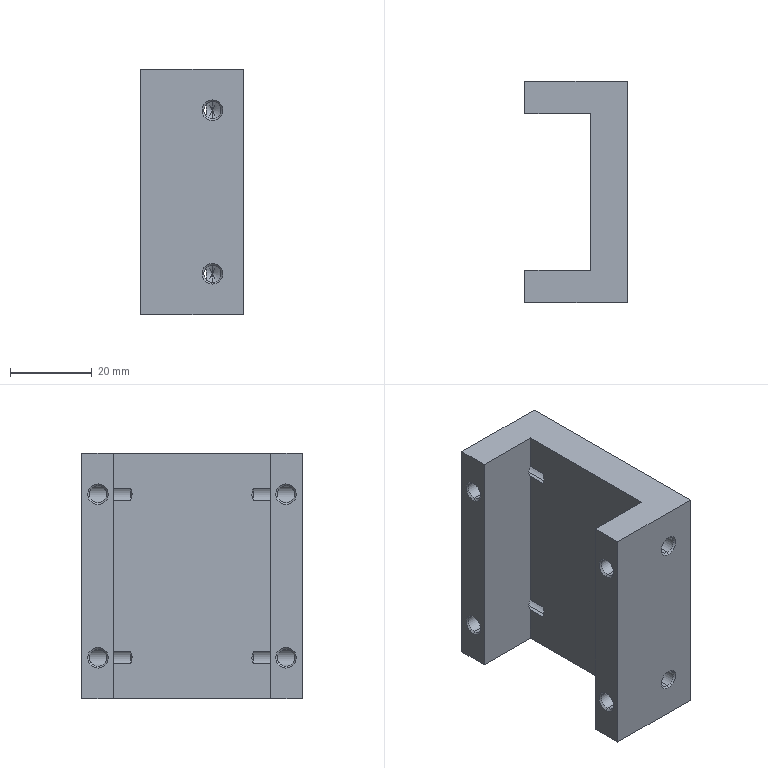Component | SolidWorks | RubberHolder-1 | 1 solid | 54 faces | volume 42492 mm3 | cone 24 | cylinder 20 | plane 10 | commonest cylinder face diameters 4.2 x20